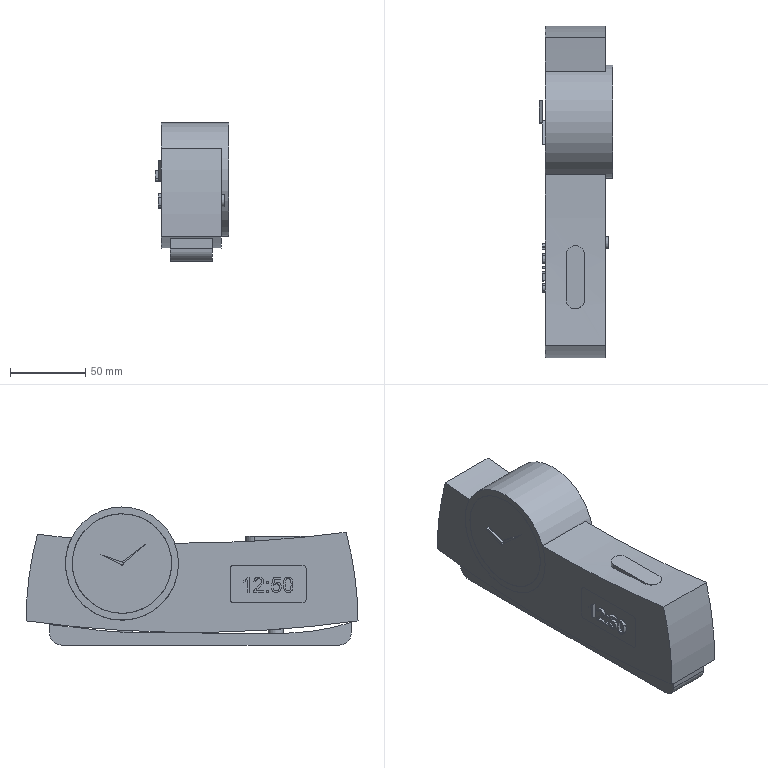Assembly | NX | mm | 11 component files | 11 solids | 155 faces | box 49 x 220 x 91.5 mm | volume 558536 mm3 | plane 84 | cylinder 40 | other 31 | commonest cylinder face diameters 4 x8 8 x6 1600 x4 10 x4 12 x4 66 x3 16 x2 75 x2
Bill of materials:
unnamed part 1 | 1 |  | Short cylinder with a circular recess in one end face, leaving a thin rim; looks like a cup.
unnamed part 2 | 1 |  | Rectangular plate-like block with rounded corners and edges. One large face is flat, and small raised features stick out from the opposite face.
unnamed part 3 | 1 |  | Constant-thickness strip with a long, tapering outline: one end is rounded and the other narrows to a sharp point, like a sliver or wedge.
unnamed part 4 | 1 |  | Long bar with a gently concave top surface, rounded lower edges at the ends, and two small short cylindrical bosses on top.
unnamed part 5 | 1 |  | Arc-shaped block with a large semicircular cutout open at one end of the top, an elongated slot through the top face, and three small holes on the front face.
unnamed part 6 | 1 |  | Plain solid cylinder, shorter in length than its diameter, with flat ends.
unnamed part 7 | 2 |  | Solid disk with flat faces and a modest thickness compared with its diameter.
unnamed part 8 | 1 |  | Prism with an obround (stadium) outline: flat top and bottom with fully rounded ends.
unnamed part 9 | 1 |  | Very thin flat circular disk with no visible holes.
unnamed part 10 | 1 |  | Slender constant-thickness strip with a long, tapering outline: rounded at one end and narrowing to a sharp point at the other.
Mates:
1. concentric | ButtonA 2 edge | Body1 1 edge
2. concentric | Button1 1 edge | Body1 1 edge
3. concentric | Key1 1 edge | Body1 1 edge
4. concentric | Key1 1 edge | Body1 1 edge
5. concentric | ClockBase1 1 edge | Body1 1 edge
6. concentric | ClockBase1 1 edge | Body1 1 edge
7. touch align | DigitalClock1 1 face | Body1 1 face
8. touch align | DigitalClock1 1 face | Body1 1 face
9. touch align | DigitalClock1 1 face | Body1 1 face
10. concentric | ClockHand1 1 edge | Body1 1 edge
11. concentric | Dial1 1 edge | ClockHand1 1 edge
12. concentric | SecondHand1 1 edge | Dial1 1 edge
13. concentric | Clock1 1 edge | SecondHand1 1 edge
14. concentric | ButtonA 1 edge | Body1 1 edge